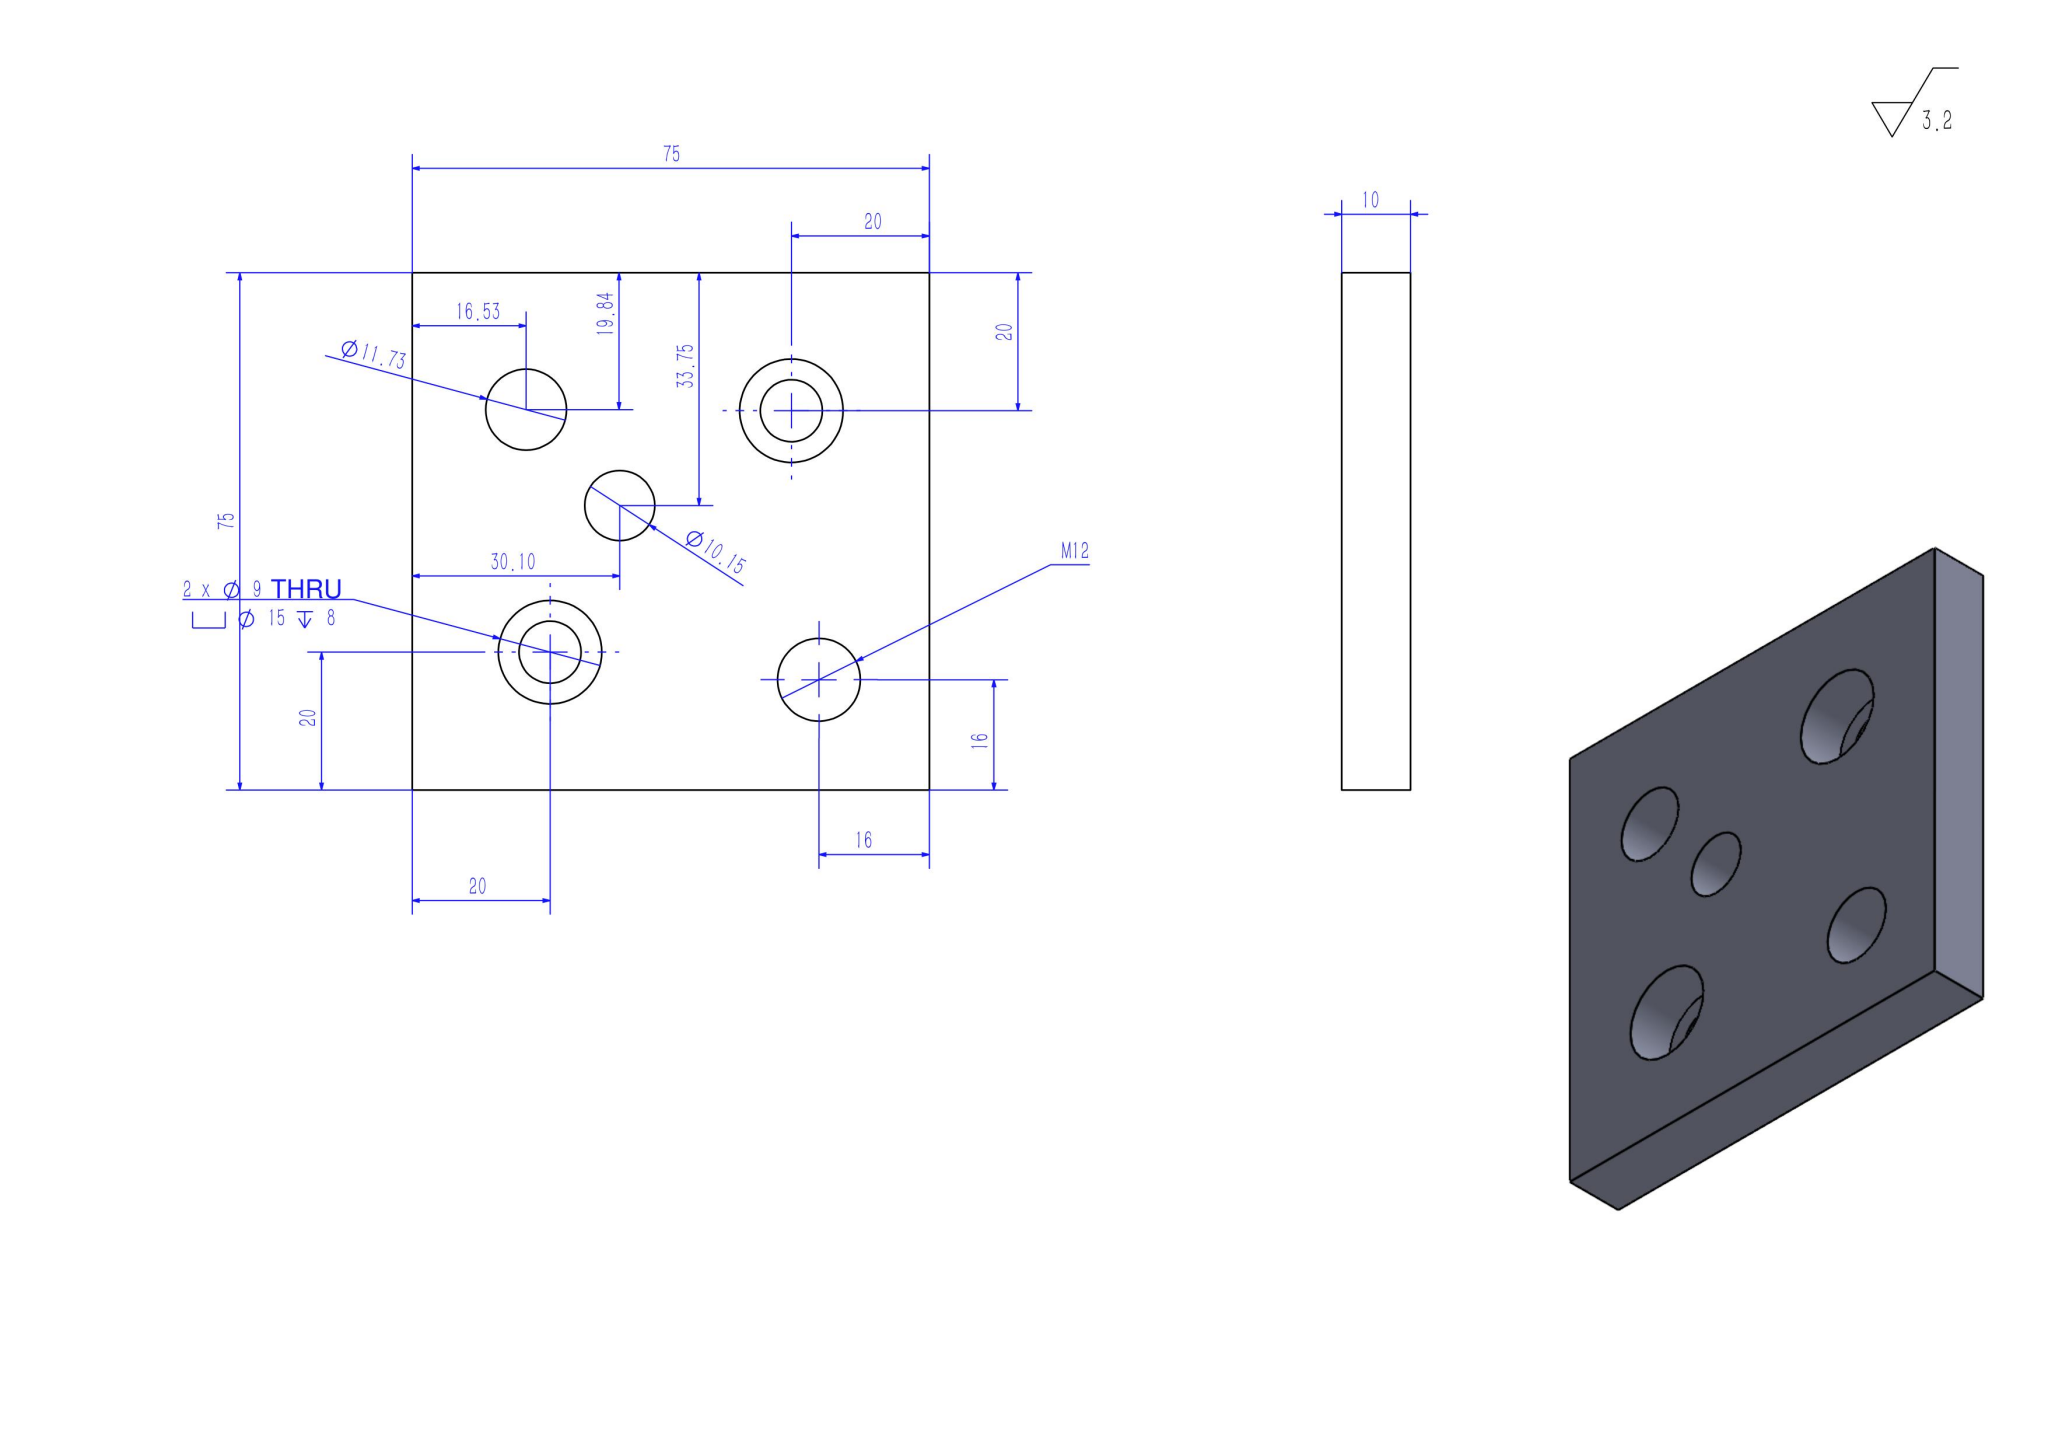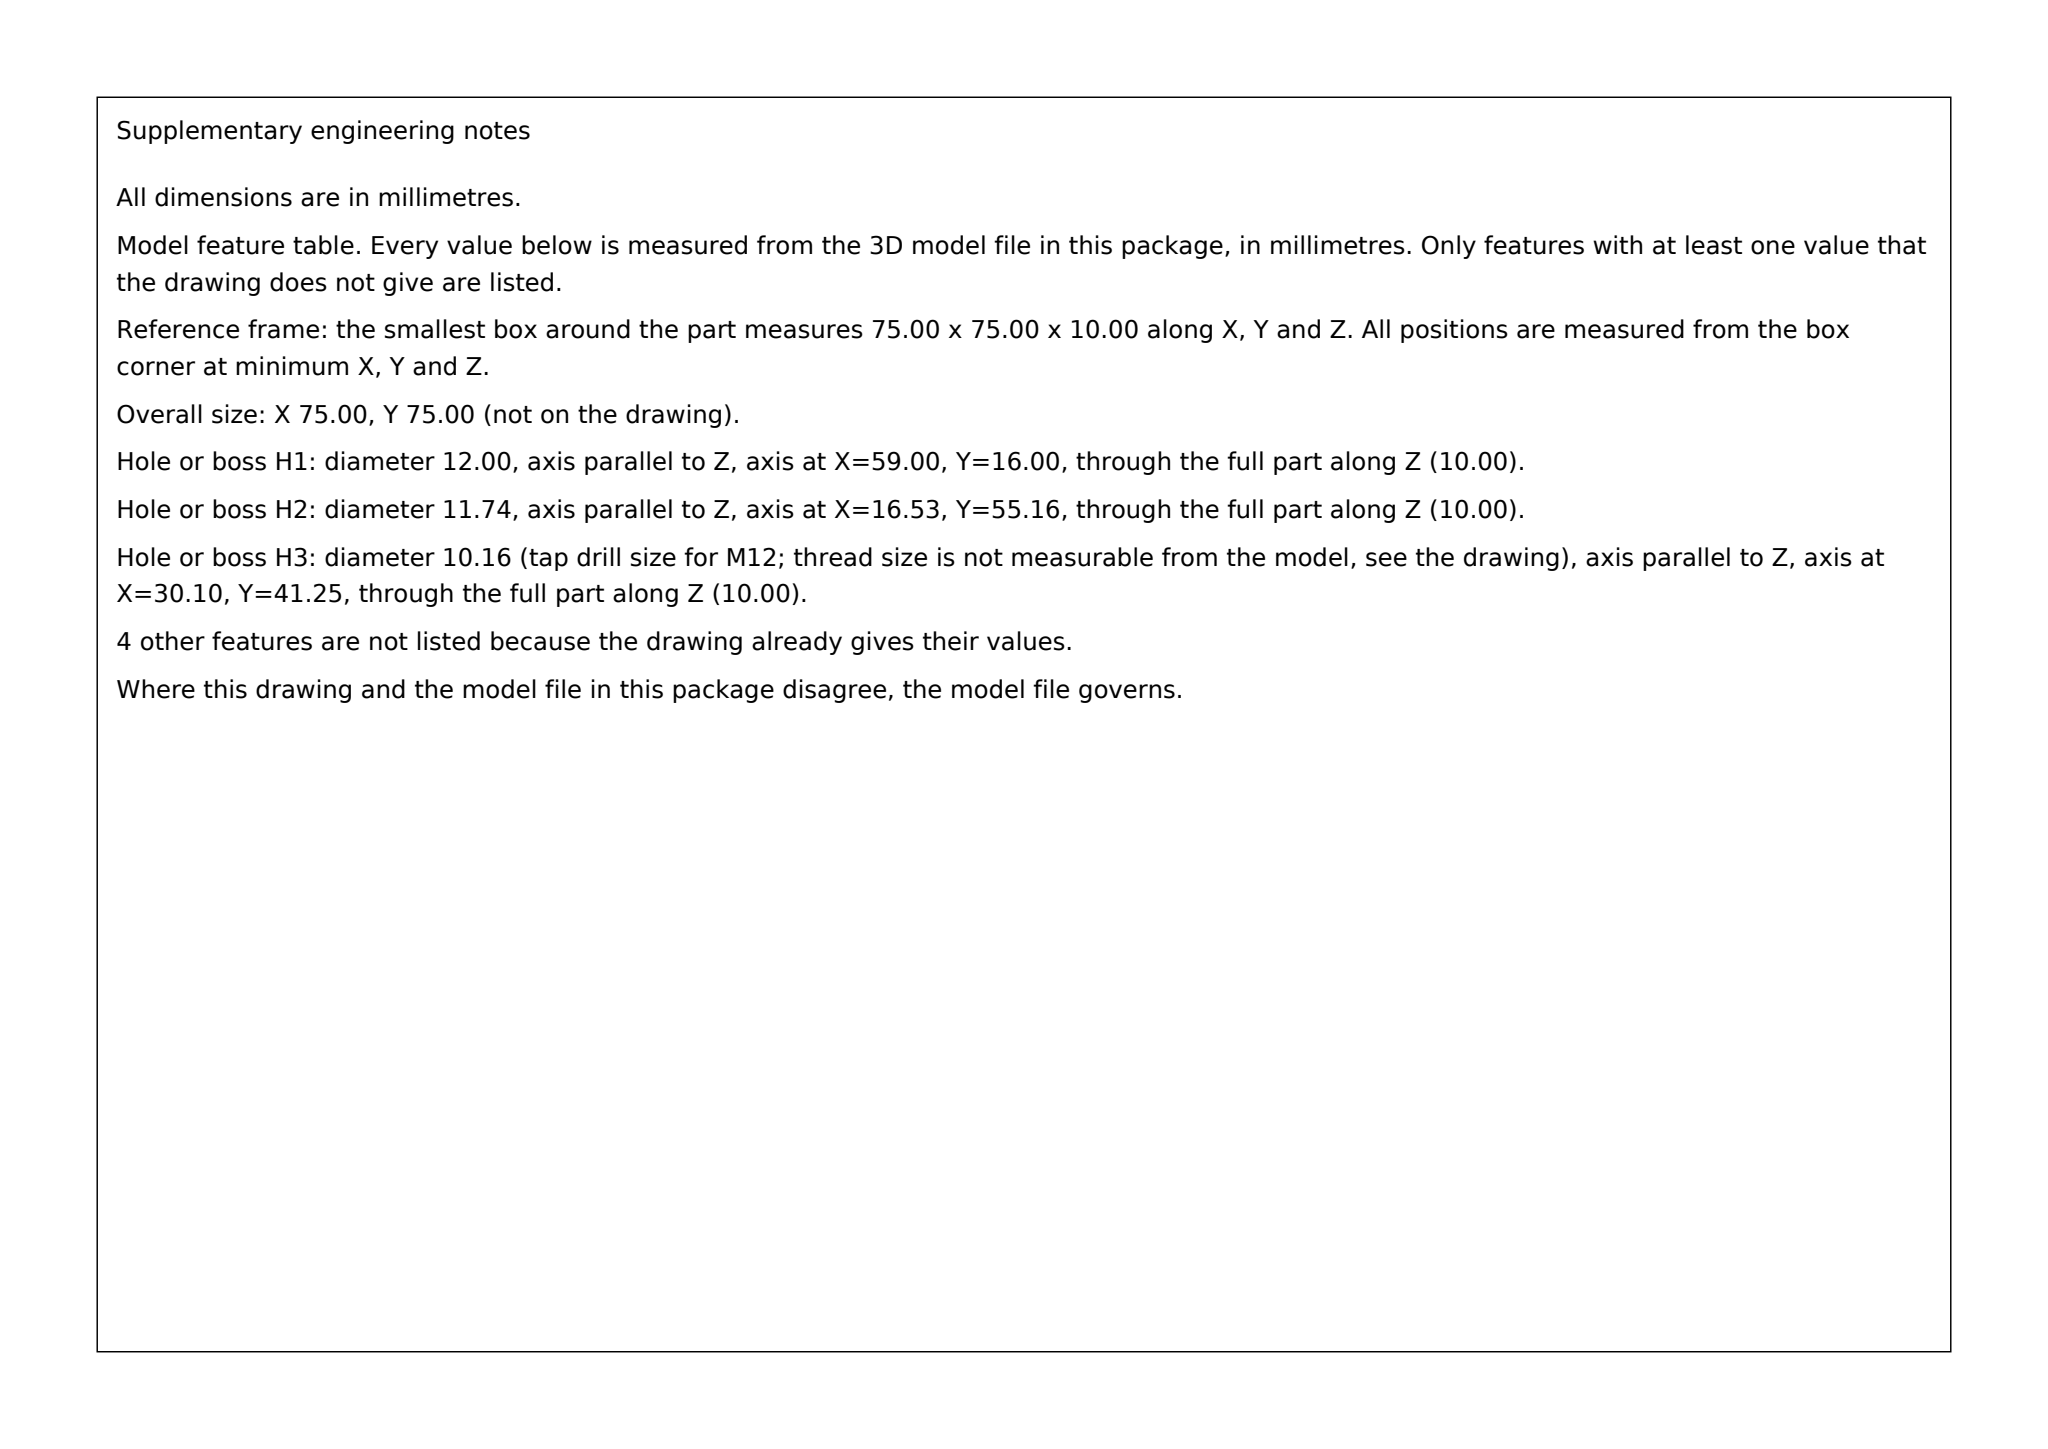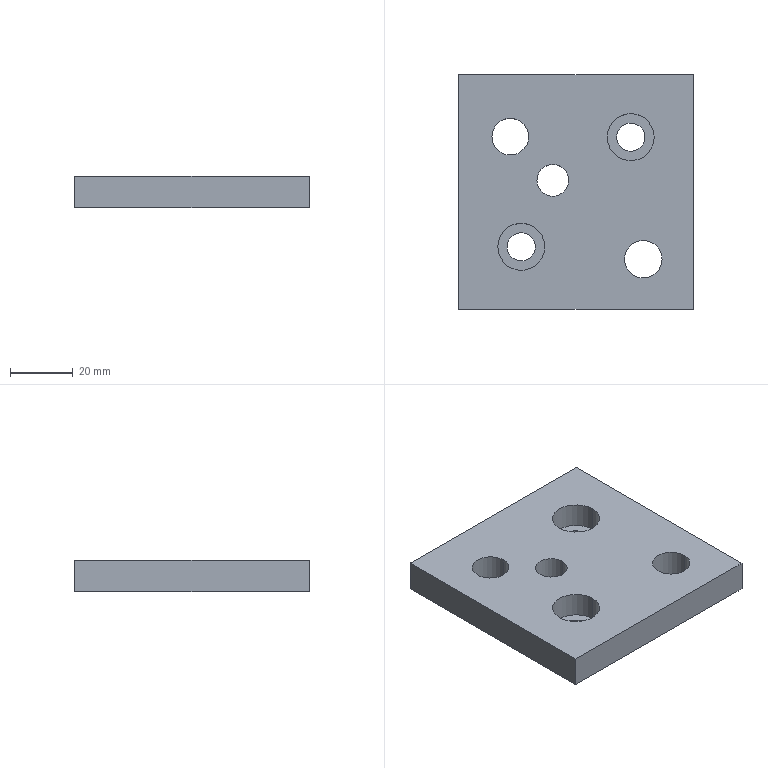Part | SolidWorks | mm | 1 solid | 22 faces | box 75 x 75 x 10 mm | volume 50146 mm3 | cylinder 14 | plane 8 | commonest cylinder face diameters 15 x4 9 x4 11.733 x2 10.155 x2 12 x2
build123d program:
from build123d import *

# Parameters (mm, degrees)
SKETCH1_W                                       = 75
SKETCH1_H                                       = 75
SKETCH1_R                                       = 6
BOSS_EXTRUDE1_DEPTH                             = 10
M8_HEX_SOCKET_HEAD_CAP_SCREW_CBORE1_D           = 9
M8_HEX_SOCKET_HEAD_CAP_SCREW_CBORE1_CBORE_D     = 15
M8_HEX_SOCKET_HEAD_CAP_SCREW_CBORE1_CBORE_DEPTH = 8
SKETCH4_R                                       = 5.867
SKETCH4_R_2                                     = 5.077
CUT_EXTRUDE1_DEPTH                              = 850


with BuildPart() as part:
    # Sketch1 → Boss-Extrude1 (new body)
    with BuildSketch(Plane.XY):
        with Locations((-942.5, 227.5)):
            Rectangle(SKETCH1_W, SKETCH1_H)
        with Locations((-921, 206)):
            Circle(SKETCH1_R, mode=Mode.SUBTRACT)
    extrude(amount=-BOSS_EXTRUDE1_DEPTH)

    # M8 Hex Socket Head Cap Screw CBORE1 (through all)
    with Locations(Plane.XY):
        with Locations((-960, 210), (-925, 245)):
            CounterBoreHole(M8_HEX_SOCKET_HEAD_CAP_SCREW_CBORE1_D / 2, M8_HEX_SOCKET_HEAD_CAP_SCREW_CBORE1_CBORE_D / 2, M8_HEX_SOCKET_HEAD_CAP_SCREW_CBORE1_CBORE_DEPTH)

    # Sketch4 → Cut-Extrude1 (cut)
    with BuildSketch(Plane.XY):
        with Locations((-963.471, 245.16)):
            Circle(SKETCH4_R)
        with Locations((-949.895, 231.253)):
            Circle(SKETCH4_R_2)
    extrude(amount=-CUT_EXTRUDE1_DEPTH, mode=Mode.SUBTRACT)


solid = part.part